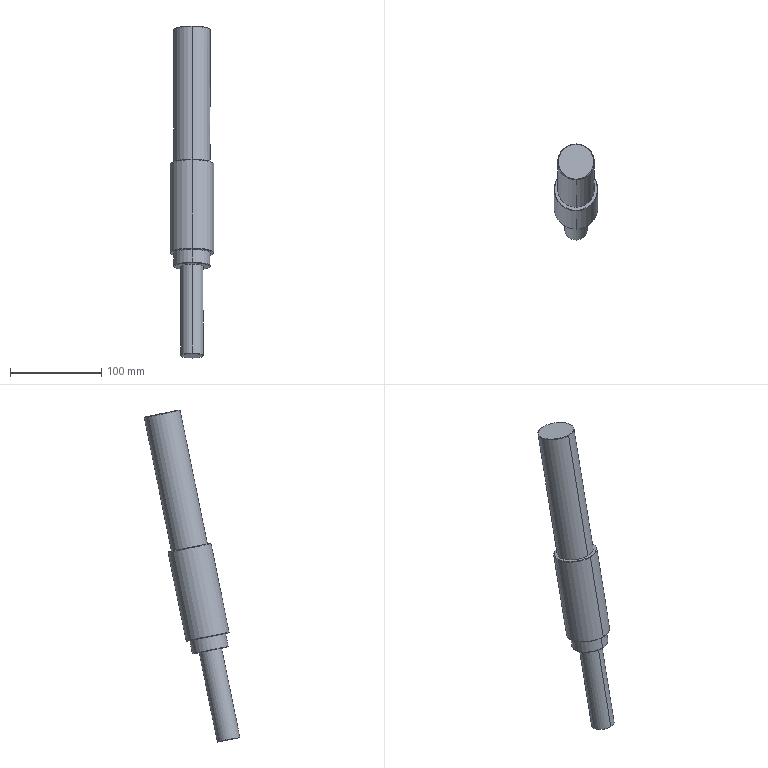Component | SolidWorks | JL001-04-01-005-1 | 1 solid | 33 faces | box 48 x 104.63 x 363.93 mm | volume 433759 mm3 | cylinder 12 | plane 11 | cone 10 | commonest cylinder face diameters 40 x4 48 x2 25 x2 10 x2 8 x2
build123d program:
from build123d import *

# Parameters (mm, degrees)
CUT_EXTRUDE1_DEPTH = 10
CHAMFER1_SIZE      = 0.5
CUT_EXTRUDE2_DEPTH = 10


with BuildPart() as part:
    # Sketch1 → Revolve1 (revolve)
    with BuildSketch(Plane.XY, mode=Mode.PRIVATE) as revolve1_sk:
        Polygon((0, 0), (0, 20), (150, 20), (150, 24), (250, 24), (250, 20), (265, 20), (265, 12.5), (365, 12.5), (365, 0), align=None)
    revolve(revolve1_sk.sketch.rotate(Axis((0, 0, 0), (1, 0, 0)), 90), axis=Axis((0, 0, 0), (1, 0, 0)))

    # Sketch2 → Cut-Extrude1 (cut)
    with BuildSketch(Plane(origin=(0, 15, 0), x_dir=(1, 0, 0), z_dir=(0, 1, 0))):
        with BuildLine():
            Line((90, 5), (125, 5))
            ThreePointArc((125, 5), (130, 0), (125, -5))
            Line((125, -5), (90, -5))
            ThreePointArc((90, -5), (85, 0), (90, 5))
        make_face()
    extrude(amount=CUT_EXTRUDE1_DEPTH, mode=Mode.SUBTRACT)

    # Chamfer1
    chamfer1_edges = [part.edges().sort_by_distance(p)[0] for p in [
        (0, 0, -20),
        (365, 0, -12.5),
        (265, 0, -20),
        (250, 0, -24),
        (150, 0, -24),
    ]]
    chamfer(chamfer1_edges, length=CHAMFER1_SIZE)

    # Sketch3 → Cut-Extrude2 (cut)
    with BuildSketch(Plane(origin=(0, 8.5, 0), x_dir=(1, 0, 0), z_dir=(0, 1, 0))):
        with BuildLine():
            Line((270, 4), (313, 4))
            ThreePointArc((313, 4), (317, 0), (313, -4))
            Line((313, -4), (270, -4))
            ThreePointArc((270, -4), (266, 0), (270, 4))
        make_face()
    extrude(amount=CUT_EXTRUDE2_DEPTH, mode=Mode.SUBTRACT)


solid = part.part

# Placed as in the assembly
solid = solid.moved(Location((0, 222.716, 261.748), (78.465, -0.0004607, -90)))
STEP:
#1=COLOUR_RGB('',0.7922,0.8196,0.9333);
#2=FILL_AREA_STYLE_COLOUR('',#1);
#3=FILL_AREA_STYLE('',(#2));
#4=SURFACE_STYLE_FILL_AREA(#3);
#5=SURFACE_SIDE_STYLE('',(#4));
#6=SURFACE_STYLE_USAGE(.BOTH.,#5);
#7=PRESENTATION_STYLE_ASSIGNMENT((#6));
#8=CARTESIAN_POINT('',(-0.,7.434,-0.07085));
#9=VERTEX_POINT('',#8);
#10=CARTESIAN_POINT('',(-0.,5.93,0.2362));
#11=VERTEX_POINT('',#10);
#12=CARTESIAN_POINT('',(-0.,6.682,0.08266));
#13=DIRECTION('',(-0.,-0.2,-0.9798));
#14=DIRECTION('',(0.,-0.9798,0.2));
#15=AXIS2_PLACEMENT_3D('',#12,#13,#14);
#16=CIRCLE('',#15,0.7677);
#17=EDGE_CURVE('',#9,#11,#16,.T.);
#18=ORIENTED_EDGE('',*,*,#17,.F.);
#19=CARTESIAN_POINT('',(-0.,7.458,-0.0555));
#20=VERTEX_POINT('',#19);
#21=CARTESIAN_POINT('',(-0.,7.458,-0.0555));
#22=DIRECTION('',(0.,0.8342,0.5514));
#23=VECTOR('',#22,39.37);
#24=LINE('',#21,#23);
#25=EDGE_CURVE('',#9,#20,#24,.T.);
#26=ORIENTED_EDGE('',*,*,#25,.T.);
#27=CARTESIAN_POINT('',(-0.,5.915,0.2594));
#28=VERTEX_POINT('',#27);
#29=CARTESIAN_POINT('',(-0.,6.686,0.1019));
#30=DIRECTION('',(0.,0.2,0.9798));
#31=DIRECTION('',(0.,-0.9798,0.2));
#32=AXIS2_PLACEMENT_3D('',#29,#30,#31);
#33=CIRCLE('',#32,0.7874);
#34=EDGE_CURVE('',#28,#20,#33,.T.);
#35=ORIENTED_EDGE('',*,*,#34,.F.);
#36=CARTESIAN_POINT('',(-0.,5.915,0.2594));
#37=DIRECTION('',(0.,-0.5514,0.8342));
#38=VECTOR('',#37,39.37);
#39=LINE('',#36,#38);
#40=EDGE_CURVE('',#11,#28,#39,.T.);
#41=ORIENTED_EDGE('',*,*,#40,.F.);
#42=EDGE_LOOP('',(#18,#26,#35,#41));
#43=FACE_OUTER_BOUND('',#42,.T.);
#44=CARTESIAN_POINT('',(-0.,6.686,0.1019));
#45=DIRECTION('',(0.,0.2,0.9798));
#46=DIRECTION('',(0.,-0.9798,0.2));
#47=AXIS2_PLACEMENT_3D('',#44,#45,#46);
#48=CONICAL_SURFACE('',#47,0.7874,0.7854);
#49=ADVANCED_FACE('',(#43),#48,.T.);
#50=CARTESIAN_POINT('',(-0.,6.358,-3.869));
#51=VERTEX_POINT('',#50);
#52=CARTESIAN_POINT('',(-0.,5.432,-3.68));
#53=VERTEX_POINT('',#52);
#54=CARTESIAN_POINT('',(-0.,5.895,-3.775));
#55=DIRECTION('',(-0.,-0.2,-0.9798));
#56=DIRECTION('',(0.,-0.9798,0.2));
#57=AXIS2_PLACEMENT_3D('',#54,#55,#56);
#58=CIRCLE('',#57,0.4724);
#59=EDGE_CURVE('',#51,#53,#58,.T.);
#60=ORIENTED_EDGE('',*,*,#59,.F.);
#61=CARTESIAN_POINT('',(-0.,6.381,-3.854));
#62=VERTEX_POINT('',#61);
#63=CARTESIAN_POINT('',(-0.,6.381,-3.854));
#64=DIRECTION('',(0.,0.8342,0.5514));
#65=VECTOR('',#64,39.37);
#66=LINE('',#63,#65);
#67=EDGE_CURVE('',#51,#62,#66,.T.);
#68=ORIENTED_EDGE('',*,*,#67,.T.);
#69=CARTESIAN_POINT('',(-0.,5.417,-3.657));
#70=VERTEX_POINT('',#69);
#71=CARTESIAN_POINT('',(-0.,5.899,-3.756));
#72=DIRECTION('',(0.,0.2,0.9798));
#73=DIRECTION('',(0.,-0.9798,0.2));
#74=AXIS2_PLACEMENT_3D('',#71,#72,#73);
#75=CIRCLE('',#74,0.4921);
#76=EDGE_CURVE('',#70,#62,#75,.T.);
#77=ORIENTED_EDGE('',*,*,#76,.F.);
#78=CARTESIAN_POINT('',(-0.,5.417,-3.657));
#79=DIRECTION('',(0.,-0.5514,0.8342));
#80=VECTOR('',#79,39.37);
#81=LINE('',#78,#80);
#82=EDGE_CURVE('',#53,#70,#81,.T.);
#83=ORIENTED_EDGE('',*,*,#82,.F.);
#84=EDGE_LOOP('',(#60,#68,#77,#83));
#85=FACE_OUTER_BOUND('',#84,.T.);
#86=CARTESIAN_POINT('',(-0.,5.899,-3.756));
#87=DIRECTION('',(0.,0.2,0.9798));
#88=DIRECTION('',(0.,-0.9798,0.2));
#89=AXIS2_PLACEMENT_3D('',#86,#87,#88);
#90=CONICAL_SURFACE('',#89,0.4921,0.7854);
#91=ADVANCED_FACE('',(#85),#90,.T.);
#92=CARTESIAN_POINT('',(-0.,8.016,10.459));
#93=VERTEX_POINT('',#92);
#94=CARTESIAN_POINT('',(-0.,9.521,10.152));
#95=VERTEX_POINT('',#94);
#96=CARTESIAN_POINT('',(-0.,8.768,10.305));
#97=DIRECTION('',(0.,0.2,0.9798));
#98=DIRECTION('',(0.,0.9798,-0.2));
#99=AXIS2_PLACEMENT_3D('',#96,#97,#98);
#100=CIRCLE('',#99,0.7677);
#101=EDGE_CURVE('',#93,#95,#100,.T.);
#102=ORIENTED_EDGE('',*,*,#101,.F.);
#103=CARTESIAN_POINT('',(-0.,7.993,10.443));
#104=VERTEX_POINT('',#103);
#105=CARTESIAN_POINT('',(-0.,8.016,10.459));
#106=DIRECTION('',(0.,-0.8342,-0.5514));
#107=VECTOR('',#106,39.37);
#108=LINE('',#105,#107);
#109=EDGE_CURVE('',#93,#104,#108,.T.);
#110=ORIENTED_EDGE('',*,*,#109,.T.);
#111=CARTESIAN_POINT('',(-0.,9.536,10.128));
#112=VERTEX_POINT('',#111);
#113=CARTESIAN_POINT('',(-0.,8.764,10.286));
#114=DIRECTION('',(-0.,-0.2,-0.9798));
#115=DIRECTION('',(0.,0.9798,-0.2));
#116=AXIS2_PLACEMENT_3D('',#113,#114,#115);
#117=CIRCLE('',#116,0.7874);
#118=EDGE_CURVE('',#112,#104,#117,.T.);
#119=ORIENTED_EDGE('',*,*,#118,.F.);
#120=CARTESIAN_POINT('',(-0.,9.521,10.152));
#121=DIRECTION('',(-0.,0.5514,-0.8342));
#122=VECTOR('',#121,39.37);
#123=LINE('',#120,#122);
#124=EDGE_CURVE('',#95,#112,#123,.T.);
#125=ORIENTED_EDGE('',*,*,#124,.F.);
#126=EDGE_LOOP('',(#102,#110,#119,#125));
#127=FACE_OUTER_BOUND('',#126,.T.);
#128=CARTESIAN_POINT('',(-0.,8.768,10.305));
#129=DIRECTION('',(-0.,-0.2,-0.9798));
#130=DIRECTION('',(0.,0.9798,-0.2));
#131=AXIS2_PLACEMENT_3D('',#128,#129,#130);
#132=CONICAL_SURFACE('',#131,0.7677,0.7854);
#133=ADVANCED_FACE('',(#127),#132,.T.);
#134=CARTESIAN_POINT('',(-0.,6.681,4.704));
#135=VERTEX_POINT('',#134);
#136=CARTESIAN_POINT('',(-0.,8.494,4.334));
#137=VERTEX_POINT('',#136);
#138=CARTESIAN_POINT('',(-0.,7.587,4.519));
#139=DIRECTION('',(0.,0.2,0.9798));
#140=DIRECTION('',(0.,0.9798,-0.2));
#141=AXIS2_PLACEMENT_3D('',#138,#139,#140);
#142=CIRCLE('',#141,0.9252);
#143=EDGE_CURVE('',#135,#137,#142,.T.);
#144=ORIENTED_EDGE('',*,*,#143,.F.);
#145=CARTESIAN_POINT('',(-0.,6.658,4.688));
#146=VERTEX_POINT('',#145);
#147=CARTESIAN_POINT('',(-0.,6.681,4.704));
#148=DIRECTION('',(0.,-0.8342,-0.5514));
#149=VECTOR('',#148,39.37);
#150=LINE('',#147,#149);
#151=EDGE_CURVE('',#135,#146,#150,.T.);
#152=ORIENTED_EDGE('',*,*,#151,.T.);
#153=CARTESIAN_POINT('',(-0.,8.509,4.311));
#154=VERTEX_POINT('',#153);
#155=CARTESIAN_POINT('',(-0.,7.584,4.499));
#156=DIRECTION('',(-0.,-0.2,-0.9798));
#157=DIRECTION('',(0.,0.9798,-0.2));
#158=AXIS2_PLACEMENT_3D('',#155,#156,#157);
#159=CIRCLE('',#158,0.9449);
#160=EDGE_CURVE('',#154,#146,#159,.T.);
#161=ORIENTED_EDGE('',*,*,#160,.F.);
#162=CARTESIAN_POINT('',(-0.,8.494,4.334));
#163=DIRECTION('',(-0.,0.5514,-0.8342));
#164=VECTOR('',#163,39.37);
#165=LINE('',#162,#164);
#166=EDGE_CURVE('',#137,#154,#165,.T.);
#167=ORIENTED_EDGE('',*,*,#166,.F.);
#168=EDGE_LOOP('',(#144,#152,#161,#167));
#169=FACE_OUTER_BOUND('',#168,.T.);
#170=CARTESIAN_POINT('',(-0.,7.587,4.519));
#171=DIRECTION('',(-0.,-0.2,-0.9798));
#172=DIRECTION('',(0.,0.9798,-0.2));
#173=AXIS2_PLACEMENT_3D('',#170,#171,#172);
#174=CONICAL_SURFACE('',#173,0.9252,0.7854);
#175=ADVANCED_FACE('',(#169),#174,.T.);
#176=CARTESIAN_POINT('',(-0.,7.707,0.4763));
#177=VERTEX_POINT('',#176);
#178=CARTESIAN_POINT('',(-0.,5.894,0.8463));
#179=VERTEX_POINT('',#178);
#180=CARTESIAN_POINT('',(-0.,6.8,0.6613));
#181=DIRECTION('',(-0.,-0.2,-0.9798));
#182=DIRECTION('',(0.,-0.9798,0.2));
#183=AXIS2_PLACEMENT_3D('',#180,#181,#182);
#184=CIRCLE('',#183,0.9252);
#185=EDGE_CURVE('',#177,#179,#184,.T.);
#186=ORIENTED_EDGE('',*,*,#185,.F.);
#187=CARTESIAN_POINT('',(-0.,7.73,0.4916));
#188=VERTEX_POINT('',#187);
#189=CARTESIAN_POINT('',(-0.,7.73,0.4916));
#190=DIRECTION('',(0.,0.8342,0.5514));
#191=VECTOR('',#190,39.37);
#192=LINE('',#189,#191);
#193=EDGE_CURVE('',#177,#188,#192,.T.);
#194=ORIENTED_EDGE('',*,*,#193,.T.);
#195=CARTESIAN_POINT('',(-0.,5.878,0.8695));
#196=VERTEX_POINT('',#195);
#197=CARTESIAN_POINT('',(-0.,6.804,0.6806));
#198=DIRECTION('',(0.,0.2,0.9798));
#199=DIRECTION('',(0.,-0.9798,0.2));
#200=AXIS2_PLACEMENT_3D('',#197,#198,#199);
#201=CIRCLE('',#200,0.9449);
#202=EDGE_CURVE('',#196,#188,#201,.T.);
#203=ORIENTED_EDGE('',*,*,#202,.F.);
#204=CARTESIAN_POINT('',(-0.,5.878,0.8695));
#205=DIRECTION('',(0.,-0.5514,0.8342));
#206=VECTOR('',#205,39.37);
#207=LINE('',#204,#206);
#208=EDGE_CURVE('',#179,#196,#207,.T.);
#209=ORIENTED_EDGE('',*,*,#208,.F.);
#210=EDGE_LOOP('',(#186,#194,#203,#209));
#211=FACE_OUTER_BOUND('',#210,.T.);
#212=CARTESIAN_POINT('',(-0.,6.804,0.6806));
#213=DIRECTION('',(0.,0.2,0.9798));
#214=DIRECTION('',(0.,-0.9798,0.2));
#215=AXIS2_PLACEMENT_3D('',#212,#213,#214);
#216=CONICAL_SURFACE('',#215,0.9449,0.7854);
#217=ADVANCED_FACE('',(#211),#216,.T.);
#218=ORIENTED_EDGE('',*,*,#34,.T.);
#219=CARTESIAN_POINT('',(-0.,7.572,0.5038));
#220=VERTEX_POINT('',#219);
#221=CARTESIAN_POINT('',(-0.,9.54,10.148));
#222=DIRECTION('',(0.,0.2,0.9798));
#223=VECTOR('',#222,39.37);
#224=LINE('',#221,#223);
#225=EDGE_CURVE('',#20,#220,#224,.T.);
#226=ORIENTED_EDGE('',*,*,#225,.T.);
#227=CARTESIAN_POINT('',(-0.,6.029,0.8187));
#228=VERTEX_POINT('',#227);
#229=CARTESIAN_POINT('',(-0.,6.8,0.6613));
#230=DIRECTION('',(0.,0.2,0.9798));
#231=DIRECTION('',(0.,-0.9798,0.2));
#232=AXIS2_PLACEMENT_3D('',#229,#230,#231);
#233=CIRCLE('',#232,0.7874);
#234=EDGE_CURVE('',#228,#220,#233,.T.);
#235=ORIENTED_EDGE('',*,*,#234,.F.);
#236=CARTESIAN_POINT('',(-0.,7.997,10.462));
#237=DIRECTION('',(0.,0.2,0.9798));
#238=VECTOR('',#237,39.37);
#239=LINE('',#236,#238);
#240=EDGE_CURVE('',#28,#228,#239,.T.);
#241=ORIENTED_EDGE('',*,*,#240,.F.);
#242=EDGE_LOOP('',(#218,#226,#235,#241));
#243=FACE_OUTER_BOUND('',#242,.T.);
#244=CARTESIAN_POINT('',(-0.,8.768,10.305));
#245=DIRECTION('',(0.,0.2,0.9798));
#246=DIRECTION('',(0.,-0.9798,0.2));
#247=AXIS2_PLACEMENT_3D('',#244,#245,#246);
#248=CYLINDRICAL_SURFACE('',#247,0.7874);
#249=ADVANCED_FACE('',(#243),#248,.T.);
#250=ORIENTED_EDGE('',*,*,#202,.T.);
#251=CARTESIAN_POINT('',(-0.,9.694,10.116));
#252=DIRECTION('',(0.,0.2,0.9798));
#253=VECTOR('',#252,39.37);
#254=LINE('',#251,#253);
#255=EDGE_CURVE('',#188,#154,#254,.T.);
#256=ORIENTED_EDGE('',*,*,#255,.T.);
#257=ORIENTED_EDGE('',*,*,#160,.T.);
#258=CARTESIAN_POINT('',(-0.,7.843,10.494));
#259=DIRECTION('',(0.,0.2,0.9798));
#260=VECTOR('',#259,39.37);
#261=LINE('',#258,#260);
#262=EDGE_CURVE('',#196,#146,#261,.T.);
#263=ORIENTED_EDGE('',*,*,#262,.F.);
#264=EDGE_LOOP('',(#250,#256,#257,#263));
#265=FACE_OUTER_BOUND('',#264,.T.);
#266=CARTESIAN_POINT('',(-0.,8.768,10.305));
#267=DIRECTION('',(0.,0.2,0.9798));
#268=DIRECTION('',(0.,-0.9798,0.2));
#269=AXIS2_PLACEMENT_3D('',#266,#267,#268);
#270=CYLINDRICAL_SURFACE('',#269,0.9449);
#271=ADVANCED_FACE('',(#265),#270,.T.);
#272=CARTESIAN_POINT('',(0.7624,8.253,6.794));
#273=VERTEX_POINT('',#272);
#274=CARTESIAN_POINT('',(0.7624,7.867,6.873));
#275=VERTEX_POINT('',#274);
#276=CARTESIAN_POINT('',(0.7624,8.253,6.794));
#277=CARTESIAN_POINT('',(0.7624,8.255,6.807));
#278=CARTESIAN_POINT('',(0.7627,8.257,6.82));
#279=CARTESIAN_POINT('',(0.764,8.257,6.845));
#280=CARTESIAN_POINT('',(0.765,8.256,6.858));
#281=CARTESIAN_POINT('',(0.7673,8.251,6.884));
#282=CARTESIAN_POINT('',(0.7687,8.247,6.896));
#283=CARTESIAN_POINT('',(0.7717,8.237,6.92));
#284=CARTESIAN_POINT('',(0.7734,8.231,6.931));
#285=CARTESIAN_POINT('',(0.7766,8.217,6.952));
#286=CARTESIAN_POINT('',(0.7782,8.209,6.962));
#287=CARTESIAN_POINT('',(0.7813,8.191,6.981));
#288=CARTESIAN_POINT('',(0.7826,8.181,6.989));
#289=CARTESIAN_POINT('',(0.7843,8.165,7.));
#290=CARTESIAN_POINT('',(0.7849,8.159,7.003));
#291=CARTESIAN_POINT('',(0.7858,8.148,7.009));
#292=CARTESIAN_POINT('',(0.7861,8.142,7.012));
#293=CARTESIAN_POINT('',(0.7871,8.124,7.02));
#294=CARTESIAN_POINT('',(0.7874,8.112,7.024));
#295=CARTESIAN_POINT('',(0.7874,8.087,7.029));
#296=CARTESIAN_POINT('',(0.7871,8.074,7.03));
#297=CARTESIAN_POINT('',(0.7858,8.048,7.03));
#298=CARTESIAN_POINT('',(0.7849,8.035,7.029));
#299=CARTESIAN_POINT('',(0.7826,8.01,7.024));
#300=CARTESIAN_POINT('',(0.7813,7.997,7.02));
#301=CARTESIAN_POINT('',(0.7783,7.974,7.011));
#302=CARTESIAN_POINT('',(0.7766,7.962,7.005));
#303=CARTESIAN_POINT('',(0.7734,7.941,6.99));
#304=CARTESIAN_POINT('',(0.7718,7.931,6.982));
#305=CARTESIAN_POINT('',(0.7687,7.912,6.964));
#306=CARTESIAN_POINT('',(0.7673,7.904,6.954));
#307=CARTESIAN_POINT('',(0.765,7.89,6.933));
#308=CARTESIAN_POINT('',(0.764,7.884,6.922));
#309=CARTESIAN_POINT('',(0.7627,7.873,6.898));
#310=CARTESIAN_POINT('',(0.7624,7.87,6.885));
#311=CARTESIAN_POINT('',(0.7624,7.867,6.873));
#312=B_SPLINE_CURVE_WITH_KNOTS('',3,(#276,#277,#278,#279,#280,#281,#282,#283,#284,#285,#286,#287,#288,#289,#290,#291,#292,#293,#294,#295,#296,#297,#298,#299,#300,#301,#302,#303,#304,#305,#306,#307,#308,#309,#310,#311),.UNSPECIFIED.,.F.,.F.,(4,2,2,2,2,2,2,2,2,2,2,2,2,2,2,2,2,4),(0.,0.0009806,0.001961,0.002942,0.003922,0.004903,0.005884,0.006374,0.006864,0.007845,0.008826,0.009806,0.01079,0.01177,0.01275,0.01373,0.01471,0.01569),.UNSPECIFIED.);
#313=EDGE_CURVE('',#273,#275,#312,.T.);
#314=ORIENTED_EDGE('',*,*,#313,.F.);
#315=CARTESIAN_POINT('',(0.7624,7.977,5.444));
#316=VERTEX_POINT('',#315);
#317=CARTESIAN_POINT('',(0.7624,8.961,10.266));
#318=DIRECTION('',(0.,0.2,0.9798));
#319=VECTOR('',#318,39.37);
#320=LINE('',#317,#319);
#321=EDGE_CURVE('',#316,#273,#320,.T.);
#322=ORIENTED_EDGE('',*,*,#321,.F.);
#323=CARTESIAN_POINT('',(0.7624,7.591,5.523));
#324=VERTEX_POINT('',#323);
#325=CARTESIAN_POINT('',(0.7624,7.591,5.523));
#326=CARTESIAN_POINT('',(0.7624,7.589,5.51));
#327=CARTESIAN_POINT('',(0.7627,7.588,5.497));
#328=CARTESIAN_POINT('',(0.764,7.587,5.471));
#329=CARTESIAN_POINT('',(0.765,7.589,5.458));
#330=CARTESIAN_POINT('',(0.7673,7.594,5.433));
#331=CARTESIAN_POINT('',(0.7687,7.597,5.421));
#332=CARTESIAN_POINT('',(0.7717,7.607,5.397));
#333=CARTESIAN_POINT('',(0.7734,7.613,5.385));
#334=CARTESIAN_POINT('',(0.7766,7.627,5.364));
#335=CARTESIAN_POINT('',(0.7782,7.635,5.354));
#336=CARTESIAN_POINT('',(0.7813,7.653,5.336));
#337=CARTESIAN_POINT('',(0.7826,7.663,5.327));
#338=CARTESIAN_POINT('',(0.7843,7.679,5.317));
#339=CARTESIAN_POINT('',(0.7849,7.685,5.313));
#340=CARTESIAN_POINT('',(0.7858,7.696,5.307));
#341=CARTESIAN_POINT('',(0.7861,7.702,5.304));
#342=CARTESIAN_POINT('',(0.7871,7.72,5.297));
#343=CARTESIAN_POINT('',(0.7874,7.732,5.293));
#344=CARTESIAN_POINT('',(0.7874,7.757,5.288));
#345=CARTESIAN_POINT('',(0.7871,7.771,5.286));
#346=CARTESIAN_POINT('',(0.7858,7.796,5.286));
#347=CARTESIAN_POINT('',(0.7849,7.809,5.287));
#348=CARTESIAN_POINT('',(0.7826,7.834,5.292));
#349=CARTESIAN_POINT('',(0.7813,7.847,5.296));
#350=CARTESIAN_POINT('',(0.7783,7.871,5.306));
#351=CARTESIAN_POINT('',(0.7766,7.882,5.312));
#352=CARTESIAN_POINT('',(0.7734,7.904,5.326));
#353=CARTESIAN_POINT('',(0.7718,7.913,5.334));
#354=CARTESIAN_POINT('',(0.7687,7.932,5.352));
#355=CARTESIAN_POINT('',(0.7673,7.94,5.362));
#356=CARTESIAN_POINT('',(0.765,7.954,5.383));
#357=CARTESIAN_POINT('',(0.764,7.961,5.395));
#358=CARTESIAN_POINT('',(0.7627,7.971,5.418));
#359=CARTESIAN_POINT('',(0.7624,7.975,5.431));
#360=CARTESIAN_POINT('',(0.7624,7.977,5.444));
#361=B_SPLINE_CURVE_WITH_KNOTS('',3,(#325,#326,#327,#328,#329,#330,#331,#332,#333,#334,#335,#336,#337,#338,#339,#340,#341,#342,#343,#344,#345,#346,#347,#348,#349,#350,#351,#352,#353,#354,#355,#356,#357,#358,#359,#360),.UNSPECIFIED.,.F.,.F.,(4,2,2,2,2,2,2,2,2,2,2,2,2,2,2,2,2,4),(0.,0.0009806,0.001961,0.002942,0.003922,0.004903,0.005884,0.006374,0.006864,0.007845,0.008826,0.009806,0.01079,0.01177,0.01275,0.01373,0.01471,0.01569),.UNSPECIFIED.);
#362=EDGE_CURVE('',#324,#316,#361,.T.);
#363=ORIENTED_EDGE('',*,*,#362,.F.);
#364=CARTESIAN_POINT('',(0.7624,8.575,10.344));
#365=DIRECTION('',(-0.,-0.2,-0.9798));
#366=VECTOR('',#365,39.37);
#367=LINE('',#364,#366);
#368=EDGE_CURVE('',#275,#324,#367,.T.);
#369=ORIENTED_EDGE('',*,*,#368,.F.);
#370=EDGE_LOOP('',(#314,#322,#363,#369));
#371=FACE_BOUND('',#370,.T.);
#372=CARTESIAN_POINT('',(-0.,6.816,4.676));
#373=VERTEX_POINT('',#372);
#374=CARTESIAN_POINT('',(-0.,8.359,4.361));
#375=VERTEX_POINT('',#374);
#376=CARTESIAN_POINT('',(-0.,7.587,4.519));
#377=DIRECTION('',(0.,0.2,0.9798));
#378=DIRECTION('',(0.,-0.9798,0.2));
#379=AXIS2_PLACEMENT_3D('',#376,#377,#378);
#380=CIRCLE('',#379,0.7874);
#381=EDGE_CURVE('',#373,#375,#380,.T.);
#382=ORIENTED_EDGE('',*,*,#381,.T.);
#383=CARTESIAN_POINT('',(-0.,9.54,10.148));
#384=DIRECTION('',(0.,0.2,0.9798));
#385=VECTOR('',#384,39.37);
#386=LINE('',#383,#385);
#387=EDGE_CURVE('',#375,#112,#386,.T.);
#388=ORIENTED_EDGE('',*,*,#387,.T.);
#389=ORIENTED_EDGE('',*,*,#118,.T.);
#390=CARTESIAN_POINT('',(-0.,7.997,10.462));
#391=DIRECTION('',(0.,0.2,0.9798));
#392=VECTOR('',#391,39.37);
#393=LINE('',#390,#392);
#394=EDGE_CURVE('',#373,#104,#393,.T.);
#395=ORIENTED_EDGE('',*,*,#394,.F.);
#396=EDGE_LOOP('',(#382,#388,#389,#395));
#397=FACE_OUTER_BOUND('',#396,.T.);
#398=CARTESIAN_POINT('',(-0.,8.768,10.305));
#399=DIRECTION('',(0.,0.2,0.9798));
#400=DIRECTION('',(0.,-0.9798,0.2));
#401=AXIS2_PLACEMENT_3D('',#398,#399,#400);
#402=CYLINDRICAL_SURFACE('',#401,0.7874);
#403=ADVANCED_FACE('',(#371,#397),#402,.T.);
#404=CARTESIAN_POINT('',(0.4662,6.797,-0.1417));
#405=VERTEX_POINT('',#404);
#406=CARTESIAN_POINT('',(0.4662,6.489,-0.07872));
#407=VERTEX_POINT('',#406);
#408=CARTESIAN_POINT('',(0.4662,6.797,-0.1417));
#409=CARTESIAN_POINT('',(0.4662,6.799,-0.1314));
#410=CARTESIAN_POINT('',(0.4666,6.8,-0.1212));
#411=CARTESIAN_POINT('',(0.4679,6.8,-0.1005));
#412=CARTESIAN_POINT('',(0.4689,6.799,-0.0901));
#413=CARTESIAN_POINT('',(0.4714,6.795,-0.06987));
#414=CARTESIAN_POINT('',(0.4728,6.792,-0.06007));
#415=CARTESIAN_POINT('',(0.476,6.785,-0.04107));
#416=CARTESIAN_POINT('',(0.4777,6.78,-0.03189));
#417=CARTESIAN_POINT('',(0.481,6.769,-0.01488));
#418=CARTESIAN_POINT('',(0.4827,6.762,-0.00694));
#419=CARTESIAN_POINT('',(0.4858,6.748,0.007784));
#420=CARTESIAN_POINT('',(0.4872,6.74,0.01434));
#421=CARTESIAN_POINT('',(0.4896,6.723,0.02585));
#422=CARTESIAN_POINT('',(0.4905,6.714,0.03085));
#423=CARTESIAN_POINT('',(0.4918,6.694,0.03892));
#424=CARTESIAN_POINT('',(0.4921,6.685,0.04197));
#425=CARTESIAN_POINT('',(0.4921,6.664,0.04613));
#426=CARTESIAN_POINT('',(0.4918,6.654,0.04722));
#427=CARTESIAN_POINT('',(0.4905,6.633,0.04731));
#428=CARTESIAN_POINT('',(0.4896,6.623,0.04635));
#429=CARTESIAN_POINT('',(0.4872,6.603,0.04239));
#430=CARTESIAN_POINT('',(0.4858,6.593,0.03941));
#431=CARTESIAN_POINT('',(0.4827,6.574,0.03168));
#432=CARTESIAN_POINT('',(0.4811,6.565,0.02684));
#433=CARTESIAN_POINT('',(0.4777,6.547,0.01553));
#434=CARTESIAN_POINT('',(0.476,6.54,0.009109));
#435=CARTESIAN_POINT('',(0.4729,6.525,-0.00526));
#436=CARTESIAN_POINT('',(0.4714,6.518,-0.01329));
#437=CARTESIAN_POINT('',(0.4689,6.507,-0.03028));
#438=CARTESIAN_POINT('',(0.468,6.502,-0.03929));
#439=CARTESIAN_POINT('',(0.4666,6.494,-0.05841));
#440=CARTESIAN_POINT('',(0.4662,6.491,-0.06846));
#441=CARTESIAN_POINT('',(0.4662,6.489,-0.07872));
#442=B_SPLINE_CURVE_WITH_KNOTS('',3,(#408,#409,#410,#411,#412,#413,#414,#415,#416,#417,#418,#419,#420,#421,#422,#423,#424,#425,#426,#427,#428,#429,#430,#431,#432,#433,#434,#435,#436,#437,#438,#439,#440,#441),.UNSPECIFIED.,.F.,.F.,(4,2,2,2,2,2,2,2,2,2,2,2,2,2,2,2,4),(0.,0.0007865,0.001573,0.00236,0.003146,0.003933,0.004719,0.005506,0.006292,0.007079,0.007865,0.008652,0.009438,0.01022,0.01101,0.0118,0.01258),.UNSPECIFIED.);
#443=EDGE_CURVE('',#405,#407,#442,.T.);
#444=ORIENTED_EDGE('',*,*,#443,.F.);
#445=CARTESIAN_POINT('',(0.4662,6.459,-1.8));
#446=VERTEX_POINT('',#445);
#447=CARTESIAN_POINT('',(0.4662,8.923,10.274));
#448=DIRECTION('',(0.,0.2,0.9798));
#449=VECTOR('',#448,39.37);
#450=LINE('',#447,#449);
#451=EDGE_CURVE('',#446,#405,#450,.T.);
#452=ORIENTED_EDGE('',*,*,#451,.F.);
#453=CARTESIAN_POINT('',(0.4662,6.15,-1.737));
#454=VERTEX_POINT('',#453);
#455=CARTESIAN_POINT('',(0.4662,6.15,-1.737));
#456=CARTESIAN_POINT('',(0.4662,6.148,-1.748));
#457=CARTESIAN_POINT('',(0.4666,6.147,-1.758));
#458=CARTESIAN_POINT('',(0.4679,6.147,-1.779));
#459=CARTESIAN_POINT('',(0.4689,6.148,-1.789));
#460=CARTESIAN_POINT('',(0.4714,6.152,-1.809));
#461=CARTESIAN_POINT('',(0.4728,6.155,-1.819));
#462=CARTESIAN_POINT('',(0.476,6.162,-1.838));
#463=CARTESIAN_POINT('',(0.4777,6.167,-1.847));
#464=CARTESIAN_POINT('',(0.481,6.179,-1.864));
#465=CARTESIAN_POINT('',(0.4827,6.185,-1.872));
#466=CARTESIAN_POINT('',(0.4858,6.199,-1.887));
#467=CARTESIAN_POINT('',(0.4872,6.207,-1.893));
#468=CARTESIAN_POINT('',(0.4896,6.224,-1.905));
#469=CARTESIAN_POINT('',(0.4905,6.234,-1.91));
#470=CARTESIAN_POINT('',(0.4918,6.253,-1.918));
#471=CARTESIAN_POINT('',(0.4921,6.263,-1.921));
#472=CARTESIAN_POINT('',(0.4921,6.283,-1.925));
#473=CARTESIAN_POINT('',(0.4918,6.293,-1.926));
#474=CARTESIAN_POINT('',(0.4905,6.314,-1.926));
#475=CARTESIAN_POINT('',(0.4896,6.324,-1.925));
#476=CARTESIAN_POINT('',(0.4872,6.345,-1.922));
#477=CARTESIAN_POINT('',(0.4858,6.354,-1.919));
#478=CARTESIAN_POINT('',(0.4827,6.373,-1.911));
#479=CARTESIAN_POINT('',(0.4811,6.383,-1.906));
#480=CARTESIAN_POINT('',(0.4777,6.4,-1.895));
#481=CARTESIAN_POINT('',(0.476,6.408,-1.888));
#482=CARTESIAN_POINT('',(0.4729,6.422,-1.874));
#483=CARTESIAN_POINT('',(0.4714,6.429,-1.866));
#484=CARTESIAN_POINT('',(0.4689,6.44,-1.849));
#485=CARTESIAN_POINT('',(0.468,6.445,-1.84));
#486=CARTESIAN_POINT('',(0.4666,6.453,-1.821));
#487=CARTESIAN_POINT('',(0.4662,6.456,-1.811));
#488=CARTESIAN_POINT('',(0.4662,6.459,-1.8));
#489=B_SPLINE_CURVE_WITH_KNOTS('',3,(#455,#456,#457,#458,#459,#460,#461,#462,#463,#464,#465,#466,#467,#468,#469,#470,#471,#472,#473,#474,#475,#476,#477,#478,#479,#480,#481,#482,#483,#484,#485,#486,#487,#488),.UNSPECIFIED.,.F.,.F.,(4,2,2,2,2,2,2,2,2,2,2,2,2,2,2,2,4),(0.,0.0007865,0.001573,0.00236,0.003146,0.003933,0.004719,0.005506,0.006292,0.007079,0.007865,0.008652,0.009438,0.01022,0.01101,0.0118,0.01258),.UNSPECIFIED.);
#490=EDGE_CURVE('',#454,#446,#489,.T.);
#491=ORIENTED_EDGE('',*,*,#490,.F.);
#492=CARTESIAN_POINT('',(0.4662,8.614,10.337));
#493=DIRECTION('',(-0.,-0.2,-0.9798));
#494=VECTOR('',#493,39.37);
#495=LINE('',#492,#494);
#496=EDGE_CURVE('',#407,#454,#495,.T.);
#497=ORIENTED_EDGE('',*,*,#496,.F.);
#498=EDGE_LOOP('',(#444,#452,#491,#497));
#499=FACE_BOUND('',#498,.T.);
#500=ORIENTED_EDGE('',*,*,#76,.T.);
#501=CARTESIAN_POINT('',(-0.,7.164,-0.01574));
#502=VERTEX_POINT('',#501);
#503=CARTESIAN_POINT('',(-0.,9.251,10.207));
#504=DIRECTION('',(0.,0.2,0.9798));
#505=VECTOR('',#504,39.37);
#506=LINE('',#503,#505);
#507=EDGE_CURVE('',#62,#502,#506,.T.);
#508=ORIENTED_EDGE('',*,*,#507,.T.);
#509=CARTESIAN_POINT('',(-0.,6.2,0.1811));
#510=VERTEX_POINT('',#509);
#511=CARTESIAN_POINT('',(-0.,6.682,0.08266));
#512=DIRECTION('',(0.,0.2,0.9798));
#513=DIRECTION('',(0.,-0.9798,0.2));
#514=AXIS2_PLACEMENT_3D('',#511,#512,#513);
#515=CIRCLE('',#514,0.4921);
#516=EDGE_CURVE('',#510,#502,#515,.T.);
#517=ORIENTED_EDGE('',*,*,#516,.F.);
#518=CARTESIAN_POINT('',(-0.,8.286,10.403));
#519=DIRECTION('',(0.,0.2,0.9798));
#520=VECTOR('',#519,39.37);
#521=LINE('',#518,#520);
#522=EDGE_CURVE('',#70,#510,#521,.T.);
#523=ORIENTED_EDGE('',*,*,#522,.F.);
#524=EDGE_LOOP('',(#500,#508,#517,#523));
#525=FACE_OUTER_BOUND('',#524,.T.);
#526=CARTESIAN_POINT('',(-0.,8.768,10.305));
#527=DIRECTION('',(0.,0.2,0.9798));
#528=DIRECTION('',(0.,-0.9798,0.2));
#529=AXIS2_PLACEMENT_3D('',#526,#527,#528);
#530=CYLINDRICAL_SURFACE('',#529,0.4921);
#531=ADVANCED_FACE('',(#499,#525),#530,.T.);
#532=ORIENTED_EDGE('',*,*,#507,.F.);
#533=CARTESIAN_POINT('',(-0.,5.899,-3.756));
#534=DIRECTION('',(0.,0.2,0.9798));
#535=DIRECTION('',(0.,-0.9798,0.2));
#536=AXIS2_PLACEMENT_3D('',#533,#534,#535);
#537=CIRCLE('',#536,0.4921);
#538=EDGE_CURVE('',#62,#70,#537,.T.);
#539=ORIENTED_EDGE('',*,*,#538,.T.);
#540=ORIENTED_EDGE('',*,*,#522,.T.);
#541=CARTESIAN_POINT('',(-0.,6.682,0.08266));
#542=DIRECTION('',(0.,0.2,0.9798));
#543=DIRECTION('',(0.,-0.9798,0.2));
#544=AXIS2_PLACEMENT_3D('',#541,#542,#543);
#545=CIRCLE('',#544,0.4921);
#546=EDGE_CURVE('',#502,#510,#545,.T.);
#547=ORIENTED_EDGE('',*,*,#546,.F.);
#548=EDGE_LOOP('',(#532,#539,#540,#547));
#549=FACE_OUTER_BOUND('',#548,.T.);
#550=CARTESIAN_POINT('',(-0.,8.768,10.305));
#551=DIRECTION('',(0.,0.2,0.9798));
#552=DIRECTION('',(0.,-0.9798,0.2));
#553=AXIS2_PLACEMENT_3D('',#550,#551,#552);
#554=CYLINDRICAL_SURFACE('',#553,0.4921);
#555=ADVANCED_FACE('',(#549),#554,.T.);
#556=ORIENTED_EDGE('',*,*,#387,.F.);
#557=CARTESIAN_POINT('',(-0.,7.587,4.519));
#558=DIRECTION('',(0.,0.2,0.9798));
#559=DIRECTION('',(0.,-0.9798,0.2));
#560=AXIS2_PLACEMENT_3D('',#557,#558,#559);
#561=CIRCLE('',#560,0.7874);
#562=EDGE_CURVE('',#375,#373,#561,.T.);
#563=ORIENTED_EDGE('',*,*,#562,.T.);
#564=ORIENTED_EDGE('',*,*,#394,.T.);
#565=CARTESIAN_POINT('',(-0.,8.764,10.286));
#566=DIRECTION('',(-0.,-0.2,-0.9798));
#567=DIRECTION('',(0.,0.9798,-0.2));
#568=AXIS2_PLACEMENT_3D('',#565,#566,#567);
#569=CIRCLE('',#568,0.7874);
#570=EDGE_CURVE('',#104,#112,#569,.T.);
#571=ORIENTED_EDGE('',*,*,#570,.T.);
#572=EDGE_LOOP('',(#556,#563,#564,#571));
#573=FACE_OUTER_BOUND('',#572,.T.);
#574=CARTESIAN_POINT('',(-0.,8.768,10.305));
#575=DIRECTION('',(0.,0.2,0.9798));
#576=DIRECTION('',(0.,-0.9798,0.2));
#577=AXIS2_PLACEMENT_3D('',#574,#575,#576);
#578=CYLINDRICAL_SURFACE('',#577,0.7874);
#579=ADVANCED_FACE('',(#573),#578,.T.);
#580=CARTESIAN_POINT('',(-0.,8.768,10.305));
#581=DIRECTION('',(0.,0.2,0.9798));
#582=DIRECTION('',(0.,0.9798,-0.2));
#583=AXIS2_PLACEMENT_3D('',#580,#581,#582);
#584=CIRCLE('',#583,0.7677);
#585=EDGE_CURVE('',#95,#93,#584,.T.);
#586=ORIENTED_EDGE('',*,*,#585,.T.);
#587=ORIENTED_EDGE('',*,*,#101,.T.);
#588=EDGE_LOOP('',(#586,#587));
#589=FACE_OUTER_BOUND('',#588,.T.);
#590=CARTESIAN_POINT('',(-0.,8.768,10.305));
#591=DIRECTION('',(-0.,-0.2,-0.9798));
#592=DIRECTION('',(0.,0.9798,-0.2));
#593=AXIS2_PLACEMENT_3D('',#590,#591,#592);
#594=PLANE('',#593);
#595=ADVANCED_FACE('',(#589),#594,.F.);
#596=CARTESIAN_POINT('',(-0.,7.587,4.519));
#597=DIRECTION('',(0.,0.2,0.9798));
#598=DIRECTION('',(0.,0.9798,-0.2));
#599=AXIS2_PLACEMENT_3D('',#596,#597,#598);
#600=CIRCLE('',#599,0.9252);
#601=EDGE_CURVE('',#137,#135,#600,.T.);
#602=ORIENTED_EDGE('',*,*,#601,.T.);
#603=ORIENTED_EDGE('',*,*,#143,.T.);
#604=EDGE_LOOP('',(#602,#603));
#605=FACE_OUTER_BOUND('',#604,.T.);
#606=ORIENTED_EDGE('',*,*,#381,.F.);
#607=ORIENTED_EDGE('',*,*,#562,.F.);
#608=EDGE_LOOP('',(#606,#607));
#609=FACE_BOUND('',#608,.T.);
#610=CARTESIAN_POINT('',(0.7874,7.587,4.519));
#611=DIRECTION('',(-0.,-0.2,-0.9798));
#612=DIRECTION('',(0.,0.9798,-0.2));
#613=AXIS2_PLACEMENT_3D('',#610,#611,#612);
#614=PLANE('',#613);
#615=ADVANCED_FACE('',(#605,#609),#614,.F.);
#616=ORIENTED_EDGE('',*,*,#255,.F.);
#617=CARTESIAN_POINT('',(-0.,6.804,0.6806));
#618=DIRECTION('',(0.,0.2,0.9798));
#619=DIRECTION('',(0.,-0.9798,0.2));
#620=AXIS2_PLACEMENT_3D('',#617,#618,#619);
#621=CIRCLE('',#620,0.9449);
#622=EDGE_CURVE('',#188,#196,#621,.T.);
#623=ORIENTED_EDGE('',*,*,#622,.T.);
#624=ORIENTED_EDGE('',*,*,#262,.T.);
#625=CARTESIAN_POINT('',(-0.,7.584,4.499));
#626=DIRECTION('',(-0.,-0.2,-0.9798));
#627=DIRECTION('',(0.,0.9798,-0.2));
#628=AXIS2_PLACEMENT_3D('',#625,#626,#627);
#629=CIRCLE('',#628,0.9449);
#630=EDGE_CURVE('',#146,#154,#629,.T.);
#631=ORIENTED_EDGE('',*,*,#630,.T.);
#632=EDGE_LOOP('',(#616,#623,#624,#631));
#633=FACE_OUTER_BOUND('',#632,.T.);
#634=CARTESIAN_POINT('',(-0.,8.768,10.305));
#635=DIRECTION('',(0.,0.2,0.9798));
#636=DIRECTION('',(0.,-0.9798,0.2));
#637=AXIS2_PLACEMENT_3D('',#634,#635,#636);
#638=CYLINDRICAL_SURFACE('',#637,0.9449);
#639=ADVANCED_FACE('',(#633),#638,.T.);
#640=CARTESIAN_POINT('',(-0.,6.8,0.6613));
#641=DIRECTION('',(-0.,-0.2,-0.9798));
#642=DIRECTION('',(0.,-0.9798,0.2));
#643=AXIS2_PLACEMENT_3D('',#640,#641,#642);
#644=CIRCLE('',#643,0.9252);
#645=EDGE_CURVE('',#179,#177,#644,.T.);
#646=ORIENTED_EDGE('',*,*,#645,.T.);
#647=ORIENTED_EDGE('',*,*,#185,.T.);
#648=EDGE_LOOP('',(#646,#647));
#649=FACE_OUTER_BOUND('',#648,.T.);
#650=ORIENTED_EDGE('',*,*,#234,.T.);
#651=CARTESIAN_POINT('',(-0.,6.8,0.6613));
#652=DIRECTION('',(0.,0.2,0.9798));
#653=DIRECTION('',(0.,-0.9798,0.2));
#654=AXIS2_PLACEMENT_3D('',#651,#652,#653);
#655=CIRCLE('',#654,0.7874);
#656=EDGE_CURVE('',#220,#228,#655,.T.);
#657=ORIENTED_EDGE('',*,*,#656,.T.);
#658=EDGE_LOOP('',(#650,#657));
#659=FACE_BOUND('',#658,.T.);
#660=CARTESIAN_POINT('',(0.9449,6.8,0.6613));
#661=DIRECTION('',(0.,0.2,0.9798));
#662=DIRECTION('',(0.,-0.9798,0.2));
#663=AXIS2_PLACEMENT_3D('',#660,#661,#662);
#664=PLANE('',#663);
#665=ADVANCED_FACE('',(#649,#659),#664,.F.);
#666=ORIENTED_EDGE('',*,*,#225,.F.);
#667=CARTESIAN_POINT('',(-0.,6.686,0.1019));
#668=DIRECTION('',(0.,0.2,0.9798));
#669=DIRECTION('',(0.,-0.9798,0.2));
#670=AXIS2_PLACEMENT_3D('',#667,#668,#669);
#671=CIRCLE('',#670,0.7874);
#672=EDGE_CURVE('',#20,#28,#671,.T.);
#673=ORIENTED_EDGE('',*,*,#672,.T.);
#674=ORIENTED_EDGE('',*,*,#240,.T.);
#675=ORIENTED_EDGE('',*,*,#656,.F.);
#676=EDGE_LOOP('',(#666,#673,#674,#675));
#677=FACE_OUTER_BOUND('',#676,.T.);
#678=CARTESIAN_POINT('',(-0.,8.768,10.305));
#679=DIRECTION('',(0.,0.2,0.9798));
#680=DIRECTION('',(0.,-0.9798,0.2));
#681=AXIS2_PLACEMENT_3D('',#678,#679,#680);
#682=CYLINDRICAL_SURFACE('',#681,0.7874);
#683=ADVANCED_FACE('',(#677),#682,.T.);
#684=CARTESIAN_POINT('',(-0.,6.682,0.08266));
#685=DIRECTION('',(-0.,-0.2,-0.9798));
#686=DIRECTION('',(0.,-0.9798,0.2));
#687=AXIS2_PLACEMENT_3D('',#684,#685,#686);
#688=CIRCLE('',#687,0.7677);
#689=EDGE_CURVE('',#11,#9,#688,.T.);
#690=ORIENTED_EDGE('',*,*,#689,.T.);
#691=ORIENTED_EDGE('',*,*,#17,.T.);
#692=EDGE_LOOP('',(#690,#691));
#693=FACE_OUTER_BOUND('',#692,.T.);
#694=ORIENTED_EDGE('',*,*,#516,.T.);
#695=ORIENTED_EDGE('',*,*,#546,.T.);
#696=EDGE_LOOP('',(#694,#695));
#697=FACE_BOUND('',#696,.T.);
#698=CARTESIAN_POINT('',(0.7874,6.682,0.08266));
#699=DIRECTION('',(0.,0.2,0.9798));
#700=DIRECTION('',(0.,-0.9798,0.2));
#701=AXIS2_PLACEMENT_3D('',#698,#699,#700);
#702=PLANE('',#701);
#703=ADVANCED_FACE('',(#693,#697),#702,.F.);
#704=CARTESIAN_POINT('',(-0.,5.895,-3.775));
#705=DIRECTION('',(-0.,-0.2,-0.9798));
#706=DIRECTION('',(0.,-0.9798,0.2));
#707=AXIS2_PLACEMENT_3D('',#704,#705,#706);
#708=CIRCLE('',#707,0.4724);
#709=EDGE_CURVE('',#53,#51,#708,.T.);
#710=ORIENTED_EDGE('',*,*,#709,.T.);
#711=ORIENTED_EDGE('',*,*,#59,.T.);
#712=EDGE_LOOP('',(#710,#711));
#713=FACE_OUTER_BOUND('',#712,.T.);
#714=CARTESIAN_POINT('',(0.4921,5.895,-3.775));
#715=DIRECTION('',(0.,0.2,0.9798));
#716=DIRECTION('',(0.,-0.9798,0.2));
#717=AXIS2_PLACEMENT_3D('',#714,#715,#716);
#718=PLANE('',#717);
#719=ADVANCED_FACE('',(#713),#718,.F.);
#720=ORIENTED_EDGE('',*,*,#313,.T.);
#721=CARTESIAN_POINT('',(0.5906,7.867,6.873));
#722=VERTEX_POINT('',#721);
#723=CARTESIAN_POINT('',(0.9843,7.867,6.873));
#724=DIRECTION('',(-1.,0.,0.));
#725=VECTOR('',#724,39.37);
#726=LINE('',#723,#725);
#727=EDGE_CURVE('',#275,#722,#726,.T.);
#728=ORIENTED_EDGE('',*,*,#727,.T.);
#729=CARTESIAN_POINT('',(0.5906,8.253,6.794));
#730=VERTEX_POINT('',#729);
#731=CARTESIAN_POINT('',(0.5906,8.06,6.833));
#732=DIRECTION('',(1.,-0.,-0.));
#733=DIRECTION('',(0.,-0.9798,0.2));
#734=AXIS2_PLACEMENT_3D('',#731,#732,#733);
#735=CIRCLE('',#734,0.1969);
#736=EDGE_CURVE('',#730,#722,#735,.T.);
#737=ORIENTED_EDGE('',*,*,#736,.F.);
#738=CARTESIAN_POINT('',(0.9843,8.253,6.794));
#739=DIRECTION('',(-1.,0.,0.));
#740=VECTOR('',#739,39.37);
#741=LINE('',#738,#740);
#742=EDGE_CURVE('',#273,#730,#741,.T.);
#743=ORIENTED_EDGE('',*,*,#742,.F.);
#744=EDGE_LOOP('',(#720,#728,#737,#743));
#745=FACE_OUTER_BOUND('',#744,.T.);
#746=CARTESIAN_POINT('',(0.9843,8.06,6.833));
#747=DIRECTION('',(-1.,0.,0.));
#748=DIRECTION('',(0.,0.9798,-0.2));
#749=AXIS2_PLACEMENT_3D('',#746,#747,#748);
#750=CYLINDRICAL_SURFACE('',#749,0.1969);
#751=ADVANCED_FACE('',(#745),#750,.F.);
#752=ORIENTED_EDGE('',*,*,#368,.T.);
#753=CARTESIAN_POINT('',(0.5906,7.591,5.523));
#754=VERTEX_POINT('',#753);
#755=CARTESIAN_POINT('',(0.9843,7.591,5.523));
#756=DIRECTION('',(-1.,0.,0.));
#757=VECTOR('',#756,39.37);
#758=LINE('',#755,#757);
#759=EDGE_CURVE('',#324,#754,#758,.T.);
#760=ORIENTED_EDGE('',*,*,#759,.T.);
#761=CARTESIAN_POINT('',(0.5906,7.867,6.873));
#762=DIRECTION('',(-0.,-0.2,-0.9798));
#763=VECTOR('',#762,39.37);
#764=LINE('',#761,#763);
#765=EDGE_CURVE('',#722,#754,#764,.T.);
#766=ORIENTED_EDGE('',*,*,#765,.F.);
#767=ORIENTED_EDGE('',*,*,#727,.F.);
#768=EDGE_LOOP('',(#752,#760,#766,#767));
#769=FACE_OUTER_BOUND('',#768,.T.);
#770=CARTESIAN_POINT('',(0.9843,7.867,6.873));
#771=DIRECTION('',(0.,0.9798,-0.2));
#772=DIRECTION('',(0.,0.2,0.9798));
#773=AXIS2_PLACEMENT_3D('',#770,#771,#772);
#774=PLANE('',#773);
#775=ADVANCED_FACE('',(#769),#774,.T.);
#776=ORIENTED_EDGE('',*,*,#362,.T.);
#777=CARTESIAN_POINT('',(0.5906,7.977,5.444));
#778=VERTEX_POINT('',#777);
#779=CARTESIAN_POINT('',(0.9843,7.977,5.444));
#780=DIRECTION('',(-1.,0.,0.));
#781=VECTOR('',#780,39.37);
#782=LINE('',#779,#781);
#783=EDGE_CURVE('',#316,#778,#782,.T.);
#784=ORIENTED_EDGE('',*,*,#783,.T.);
#785=CARTESIAN_POINT('',(0.5906,7.784,5.483));
#786=DIRECTION('',(1.,-0.,-0.));
#787=DIRECTION('',(0.,-0.9798,0.2));
#788=AXIS2_PLACEMENT_3D('',#785,#786,#787);
#789=CIRCLE('',#788,0.1969);
#790=EDGE_CURVE('',#754,#778,#789,.T.);
#791=ORIENTED_EDGE('',*,*,#790,.F.);
#792=ORIENTED_EDGE('',*,*,#759,.F.);
#793=EDGE_LOOP('',(#776,#784,#791,#792));
#794=FACE_OUTER_BOUND('',#793,.T.);
#795=CARTESIAN_POINT('',(0.9843,7.784,5.483));
#796=DIRECTION('',(-1.,0.,0.));
#797=DIRECTION('',(0.,0.9798,-0.2));
#798=AXIS2_PLACEMENT_3D('',#795,#796,#797);
#799=CYLINDRICAL_SURFACE('',#798,0.1969);
#800=ADVANCED_FACE('',(#794),#799,.F.);
#801=ORIENTED_EDGE('',*,*,#321,.T.);
#802=ORIENTED_EDGE('',*,*,#742,.T.);
#803=CARTESIAN_POINT('',(0.5906,8.253,6.794));
#804=DIRECTION('',(0.,0.2,0.9798));
#805=VECTOR('',#804,39.37);
#806=LINE('',#803,#805);
#807=EDGE_CURVE('',#778,#730,#806,.T.);
#808=ORIENTED_EDGE('',*,*,#807,.F.);
#809=ORIENTED_EDGE('',*,*,#783,.F.);
#810=EDGE_LOOP('',(#801,#802,#808,#809));
#811=FACE_OUTER_BOUND('',#810,.T.);
#812=CARTESIAN_POINT('',(0.9843,8.253,6.794));
#813=DIRECTION('',(0.,-0.9798,0.2));
#814=DIRECTION('',(-0.,-0.2,-0.9798));
#815=AXIS2_PLACEMENT_3D('',#812,#813,#814);
#816=PLANE('',#815);
#817=ADVANCED_FACE('',(#811),#816,.T.);
#818=ORIENTED_EDGE('',*,*,#736,.T.);
#819=ORIENTED_EDGE('',*,*,#765,.T.);
#820=ORIENTED_EDGE('',*,*,#790,.T.);
#821=ORIENTED_EDGE('',*,*,#807,.T.);
#822=EDGE_LOOP('',(#818,#819,#820,#821));
#823=FACE_OUTER_BOUND('',#822,.T.);
#824=CARTESIAN_POINT('',(0.5906,8.06,6.833));
#825=DIRECTION('',(1.,-0.,-0.));
#826=DIRECTION('',(0.,-0.9798,0.2));
#827=AXIS2_PLACEMENT_3D('',#824,#825,#826);
#828=PLANE('',#827);
#829=ADVANCED_FACE('',(#823),#828,.T.);
#830=ORIENTED_EDGE('',*,*,#193,.F.);
#831=ORIENTED_EDGE('',*,*,#645,.F.);
#832=ORIENTED_EDGE('',*,*,#208,.T.);
#833=ORIENTED_EDGE('',*,*,#622,.F.);
#834=EDGE_LOOP('',(#830,#831,#832,#833));
#835=FACE_OUTER_BOUND('',#834,.T.);
#836=CARTESIAN_POINT('',(-0.,6.804,0.6806));
#837=DIRECTION('',(0.,0.2,0.9798));
#838=DIRECTION('',(0.,-0.9798,0.2));
#839=AXIS2_PLACEMENT_3D('',#836,#837,#838);
#840=CONICAL_SURFACE('',#839,0.9449,0.7854);
#841=ADVANCED_FACE('',(#835),#840,.T.);
#842=ORIENTED_EDGE('',*,*,#151,.F.);
#843=ORIENTED_EDGE('',*,*,#601,.F.);
#844=ORIENTED_EDGE('',*,*,#166,.T.);
#845=ORIENTED_EDGE('',*,*,#630,.F.);
#846=EDGE_LOOP('',(#842,#843,#844,#845));
#847=FACE_OUTER_BOUND('',#846,.T.);
#848=CARTESIAN_POINT('',(-0.,7.587,4.519));
#849=DIRECTION('',(-0.,-0.2,-0.9798));
#850=DIRECTION('',(0.,0.9798,-0.2));
#851=AXIS2_PLACEMENT_3D('',#848,#849,#850);
#852=CONICAL_SURFACE('',#851,0.9252,0.7854);
#853=ADVANCED_FACE('',(#847),#852,.T.);
#854=ORIENTED_EDGE('',*,*,#109,.F.);
#855=ORIENTED_EDGE('',*,*,#585,.F.);
#856=ORIENTED_EDGE('',*,*,#124,.T.);
#857=ORIENTED_EDGE('',*,*,#570,.F.);
#858=EDGE_LOOP('',(#854,#855,#856,#857));
#859=FACE_OUTER_BOUND('',#858,.T.);
#860=CARTESIAN_POINT('',(-0.,8.768,10.305));
#861=DIRECTION('',(-0.,-0.2,-0.9798));
#862=DIRECTION('',(0.,0.9798,-0.2));
#863=AXIS2_PLACEMENT_3D('',#860,#861,#862);
#864=CONICAL_SURFACE('',#863,0.7677,0.7854);
#865=ADVANCED_FACE('',(#859),#864,.T.);
#866=ORIENTED_EDGE('',*,*,#67,.F.);
#867=ORIENTED_EDGE('',*,*,#709,.F.);
#868=ORIENTED_EDGE('',*,*,#82,.T.);
#869=ORIENTED_EDGE('',*,*,#538,.F.);
#870=EDGE_LOOP('',(#866,#867,#868,#869));
#871=FACE_OUTER_BOUND('',#870,.T.);
#872=CARTESIAN_POINT('',(-0.,5.899,-3.756));
#873=DIRECTION('',(0.,0.2,0.9798));
#874=DIRECTION('',(0.,-0.9798,0.2));
#875=AXIS2_PLACEMENT_3D('',#872,#873,#874);
#876=CONICAL_SURFACE('',#875,0.4921,0.7854);
#877=ADVANCED_FACE('',(#871),#876,.T.);
#878=ORIENTED_EDGE('',*,*,#25,.F.);
#879=ORIENTED_EDGE('',*,*,#689,.F.);
#880=ORIENTED_EDGE('',*,*,#40,.T.);
#881=ORIENTED_EDGE('',*,*,#672,.F.);
#882=EDGE_LOOP('',(#878,#879,#880,#881));
#883=FACE_OUTER_BOUND('',#882,.T.);
#884=CARTESIAN_POINT('',(-0.,6.686,0.1019));
#885=DIRECTION('',(0.,0.2,0.9798));
#886=DIRECTION('',(0.,-0.9798,0.2));
#887=AXIS2_PLACEMENT_3D('',#884,#885,#886);
#888=CONICAL_SURFACE('',#887,0.7874,0.7854);
#889=ADVANCED_FACE('',(#883),#888,.T.);
#890=ORIENTED_EDGE('',*,*,#443,.T.);
#891=CARTESIAN_POINT('',(0.3346,6.489,-0.07872));
#892=VERTEX_POINT('',#891);
#893=CARTESIAN_POINT('',(0.7283,6.489,-0.07872));
#894=DIRECTION('',(-1.,0.,0.));
#895=VECTOR('',#894,39.37);
#896=LINE('',#893,#895);
#897=EDGE_CURVE('',#407,#892,#896,.T.);
#898=ORIENTED_EDGE('',*,*,#897,.T.);
#899=CARTESIAN_POINT('',(0.3346,6.797,-0.1417));
#900=VERTEX_POINT('',#899);
#901=CARTESIAN_POINT('',(0.3346,6.643,-0.1102));
#902=DIRECTION('',(1.,-0.,-0.));
#903=DIRECTION('',(0.,-0.9798,0.2));
#904=AXIS2_PLACEMENT_3D('',#901,#902,#903);
#905=CIRCLE('',#904,0.1575);
#906=EDGE_CURVE('',#900,#892,#905,.T.);
#907=ORIENTED_EDGE('',*,*,#906,.F.);
#908=CARTESIAN_POINT('',(0.7283,6.797,-0.1417));
#909=DIRECTION('',(-1.,0.,0.));
#910=VECTOR('',#909,39.37);
#911=LINE('',#908,#910);
#912=EDGE_CURVE('',#405,#900,#911,.T.);
#913=ORIENTED_EDGE('',*,*,#912,.F.);
#914=EDGE_LOOP('',(#890,#898,#907,#913));
#915=FACE_OUTER_BOUND('',#914,.T.);
#916=CARTESIAN_POINT('',(0.7283,6.643,-0.1102));
#917=DIRECTION('',(-1.,0.,0.));
#918=DIRECTION('',(0.,0.9798,-0.2));
#919=AXIS2_PLACEMENT_3D('',#916,#917,#918);
#920=CYLINDRICAL_SURFACE('',#919,0.1575);
#921=ADVANCED_FACE('',(#915),#920,.F.);
#922=ORIENTED_EDGE('',*,*,#496,.T.);
#923=CARTESIAN_POINT('',(0.3346,6.15,-1.737));
#924=VERTEX_POINT('',#923);
#925=CARTESIAN_POINT('',(0.7283,6.15,-1.737));
#926=DIRECTION('',(-1.,0.,0.));
#927=VECTOR('',#926,39.37);
#928=LINE('',#925,#927);
#929=EDGE_CURVE('',#454,#924,#928,.T.);
#930=ORIENTED_EDGE('',*,*,#929,.T.);
#931=CARTESIAN_POINT('',(0.3346,6.489,-0.07872));
#932=DIRECTION('',(-0.,-0.2,-0.9798));
#933=VECTOR('',#932,39.37);
#934=LINE('',#931,#933);
#935=EDGE_CURVE('',#892,#924,#934,.T.);
#936=ORIENTED_EDGE('',*,*,#935,.F.);
#937=ORIENTED_EDGE('',*,*,#897,.F.);
#938=EDGE_LOOP('',(#922,#930,#936,#937));
#939=FACE_OUTER_BOUND('',#938,.T.);
#940=CARTESIAN_POINT('',(0.7283,6.489,-0.07872));
#941=DIRECTION('',(0.,0.9798,-0.2));
#942=DIRECTION('',(0.,0.2,0.9798));
#943=AXIS2_PLACEMENT_3D('',#940,#941,#942);
#944=PLANE('',#943);
#945=ADVANCED_FACE('',(#939),#944,.T.);
#946=ORIENTED_EDGE('',*,*,#490,.T.);
#947=CARTESIAN_POINT('',(0.3346,6.459,-1.8));
#948=VERTEX_POINT('',#947);
#949=CARTESIAN_POINT('',(0.7283,6.459,-1.8));
#950=DIRECTION('',(-1.,0.,0.));
#951=VECTOR('',#950,39.37);
#952=LINE('',#949,#951);
#953=EDGE_CURVE('',#446,#948,#952,.T.);
#954=ORIENTED_EDGE('',*,*,#953,.T.);
#955=CARTESIAN_POINT('',(0.3346,6.304,-1.769));
#956=DIRECTION('',(1.,-0.,-0.));
#957=DIRECTION('',(0.,-0.9798,0.2));
#958=AXIS2_PLACEMENT_3D('',#955,#956,#957);
#959=CIRCLE('',#958,0.1575);
#960=EDGE_CURVE('',#924,#948,#959,.T.);
#961=ORIENTED_EDGE('',*,*,#960,.F.);
#962=ORIENTED_EDGE('',*,*,#929,.F.);
#963=EDGE_LOOP('',(#946,#954,#961,#962));
#964=FACE_OUTER_BOUND('',#963,.T.);
#965=CARTESIAN_POINT('',(0.7283,6.304,-1.769));
#966=DIRECTION('',(-1.,0.,0.));
#967=DIRECTION('',(0.,0.9798,-0.2));
#968=AXIS2_PLACEMENT_3D('',#965,#966,#967);
#969=CYLINDRICAL_SURFACE('',#968,0.1575);
#970=ADVANCED_FACE('',(#964),#969,.F.);
#971=ORIENTED_EDGE('',*,*,#451,.T.);
#972=ORIENTED_EDGE('',*,*,#912,.T.);
#973=CARTESIAN_POINT('',(0.3346,6.797,-0.1417));
#974=DIRECTION('',(0.,0.2,0.9798));
#975=VECTOR('',#974,39.37);
#976=LINE('',#973,#975);
#977=EDGE_CURVE('',#948,#900,#976,.T.);
#978=ORIENTED_EDGE('',*,*,#977,.F.);
#979=ORIENTED_EDGE('',*,*,#953,.F.);
#980=EDGE_LOOP('',(#971,#972,#978,#979));
#981=FACE_OUTER_BOUND('',#980,.T.);
#982=CARTESIAN_POINT('',(0.7283,6.797,-0.1417));
#983=DIRECTION('',(0.,-0.9798,0.2));
#984=DIRECTION('',(-0.,-0.2,-0.9798));
#985=AXIS2_PLACEMENT_3D('',#982,#983,#984);
#986=PLANE('',#985);
#987=ADVANCED_FACE('',(#981),#986,.T.);
#988=ORIENTED_EDGE('',*,*,#906,.T.);
#989=ORIENTED_EDGE('',*,*,#935,.T.);
#990=ORIENTED_EDGE('',*,*,#960,.T.);
#991=ORIENTED_EDGE('',*,*,#977,.T.);
#992=EDGE_LOOP('',(#988,#989,#990,#991));
#993=FACE_OUTER_BOUND('',#992,.T.);
#994=CARTESIAN_POINT('',(0.3346,6.643,-0.1102));
#995=DIRECTION('',(1.,-0.,-0.));
#996=DIRECTION('',(0.,-0.9798,0.2));
#997=AXIS2_PLACEMENT_3D('',#994,#995,#996);
#998=PLANE('',#997);
#999=ADVANCED_FACE('',(#993),#998,.T.);
#1000=CLOSED_SHELL('',(#49,#91,#133,#175,#217,#249,#271,#403,#531,#555,#579,#595,#615,#639,#665,#683,#703,#719,#751,#775,#800,#817,#829,#841,#853,#865,#877,#889,#921,#945,#970,#987,#999));
#1001=MANIFOLD_SOLID_BREP('',#1000);
#1002=STYLED_ITEM('',(#7),#1001);
#1003=(LENGTH_UNIT()NAMED_UNIT(*)SI_UNIT($,.METRE.));
#1004=LENGTH_MEASURE_WITH_UNIT(LENGTH_MEASURE(0.0254),#1003);
#1005=DIMENSIONAL_EXPONENTS(1.,0.,0.,0.,0.,0.,0.);
#1006=(CONVERSION_BASED_UNIT('',#1004)LENGTH_UNIT()NAMED_UNIT(#1005));
#1007=UNCERTAINTY_MEASURE_WITH_UNIT(LENGTH_MEASURE(0.00001),#1006,'','');
#1008=(NAMED_UNIT(*)PLANE_ANGLE_UNIT()SI_UNIT($,.RADIAN.));
#1009=(NAMED_UNIT(*)SI_UNIT($,.STERADIAN.)SOLID_ANGLE_UNIT());
#1010=(GEOMETRIC_REPRESENTATION_CONTEXT(3)GLOBAL_UNCERTAINTY_ASSIGNED_CONTEXT((#1007))GLOBAL_UNIT_ASSIGNED_CONTEXT((#1006,#1008,#1009))REPRESENTATION_CONTEXT('',''));
#1011=MECHANICAL_DESIGN_GEOMETRIC_PRESENTATION_REPRESENTATION('',(#1002),#1010);
#1012=PRESENTATION_LAYER_ASSIGNMENT('','',(#1002));
#1013=CARTESIAN_POINT('',(0.,0.,0.));
#1014=DIRECTION('',(0.,0.,1.));
#1015=DIRECTION('',(1.,0.,0.));
#1016=AXIS2_PLACEMENT_3D('',#1013,#1014,#1015);
#1017=(LENGTH_UNIT()NAMED_UNIT(*)SI_UNIT($,.METRE.));
#1018=LENGTH_MEASURE_WITH_UNIT(LENGTH_MEASURE(0.0254),#1017);
#1019=DIMENSIONAL_EXPONENTS(1.,0.,0.,0.,0.,0.,0.);
#1020=(CONVERSION_BASED_UNIT('',#1018)LENGTH_UNIT()NAMED_UNIT(#1019));
#1021=UNCERTAINTY_MEASURE_WITH_UNIT(LENGTH_MEASURE(0.00001),#1020,'','');
#1022=(NAMED_UNIT(*)PLANE_ANGLE_UNIT()SI_UNIT($,.RADIAN.));
#1023=(NAMED_UNIT(*)SI_UNIT($,.STERADIAN.)SOLID_ANGLE_UNIT());
#1024=(GEOMETRIC_REPRESENTATION_CONTEXT(3)GLOBAL_UNCERTAINTY_ASSIGNED_CONTEXT((#1021))GLOBAL_UNIT_ASSIGNED_CONTEXT((#1020,#1022,#1023))REPRESENTATION_CONTEXT('',''));
#1025=ADVANCED_BREP_SHAPE_REPRESENTATION('',(#1001,#1016),#1024);